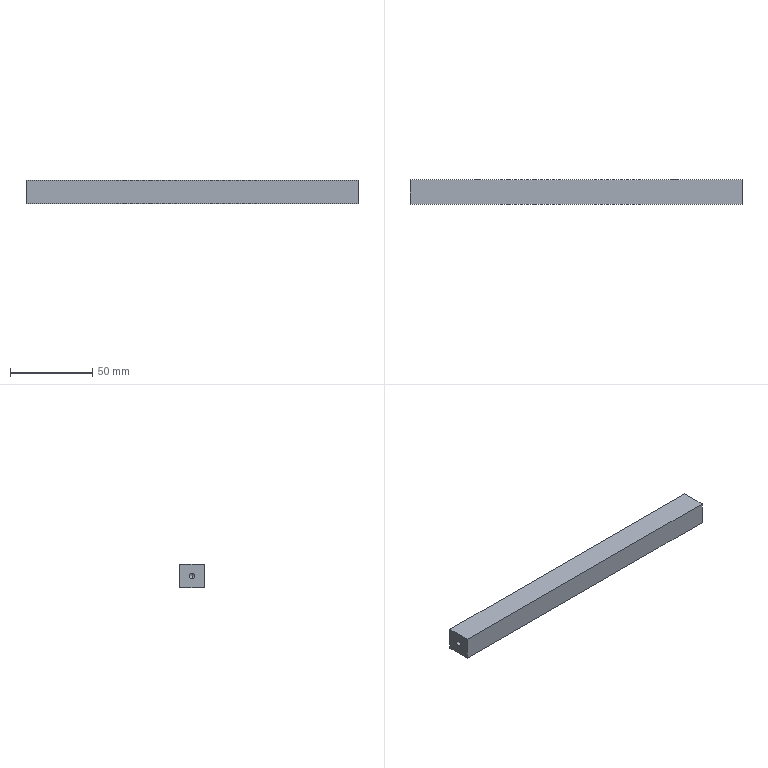CAM job | Mastercam | mm | 8 operations | part box 202 x 15 x 14
1. Facing | 12 - 12 平铣刀
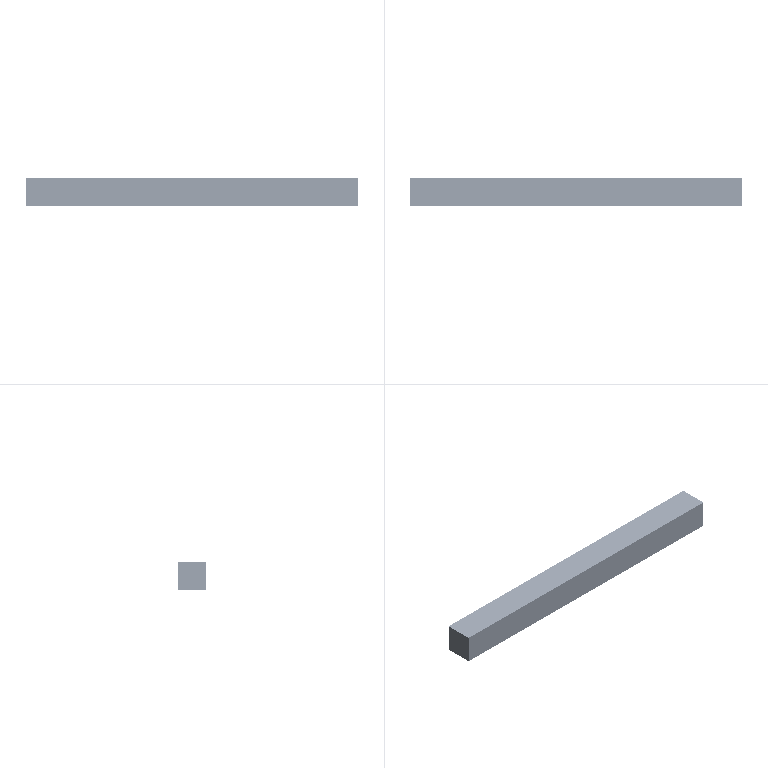2. 2D High Speed (2D Dynamic Mill) | 12 - 12 平铣刀
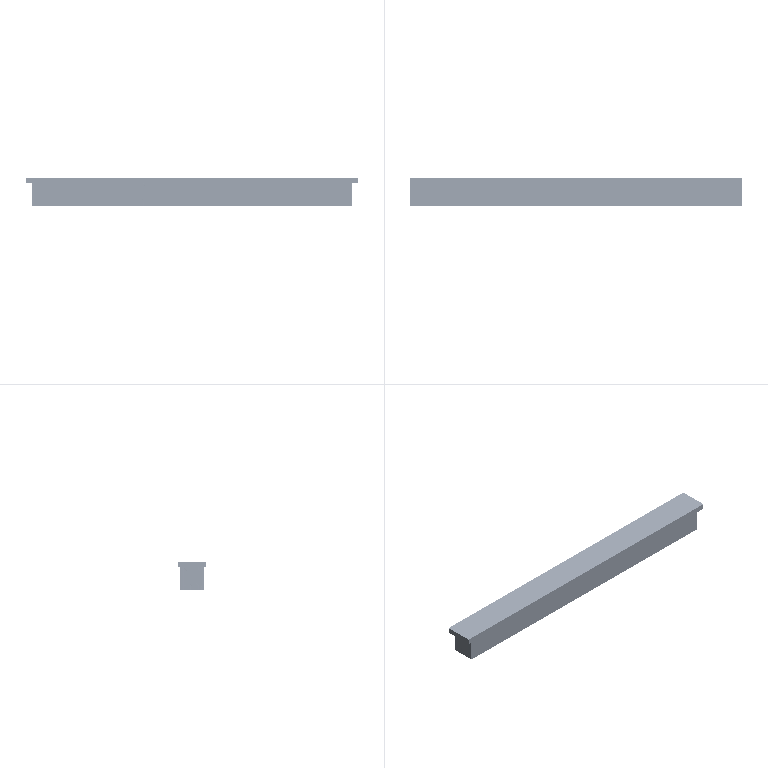3. Contour (2D) | 12 - 12 平铣刀
4. Model Chamfer | 7 - 4 倒角刀
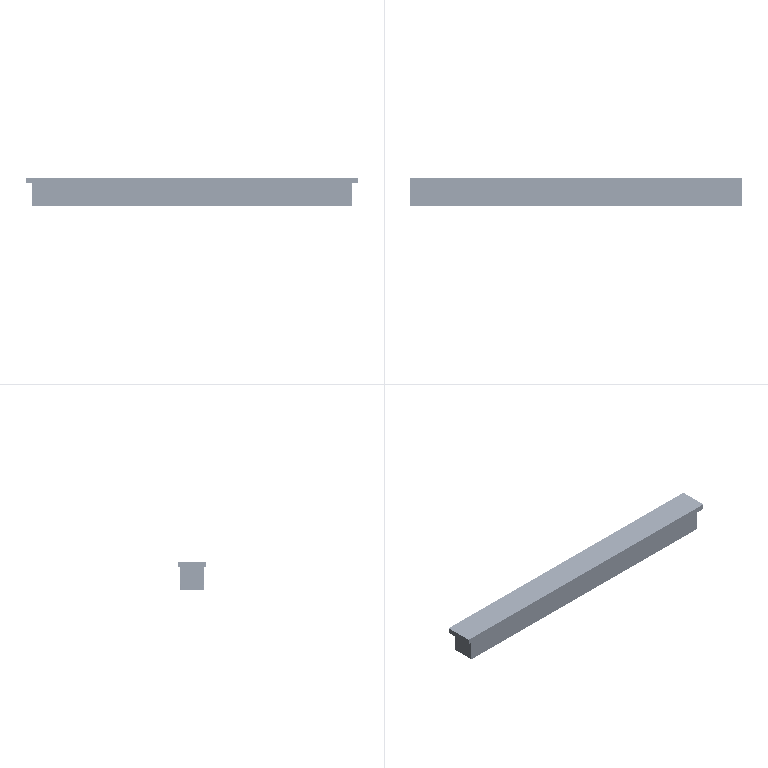5. Drill/Counterbore | 7 - 4 倒角刀
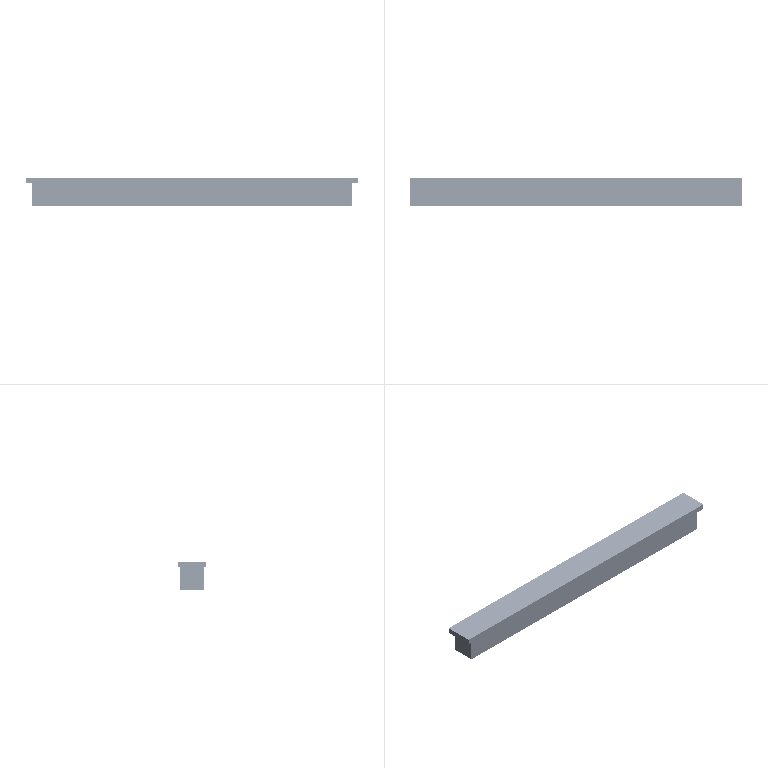6. Facing | 12 - 12 平铣刀
7. Contour (2D chamfer) | 7 - 4 倒角刀
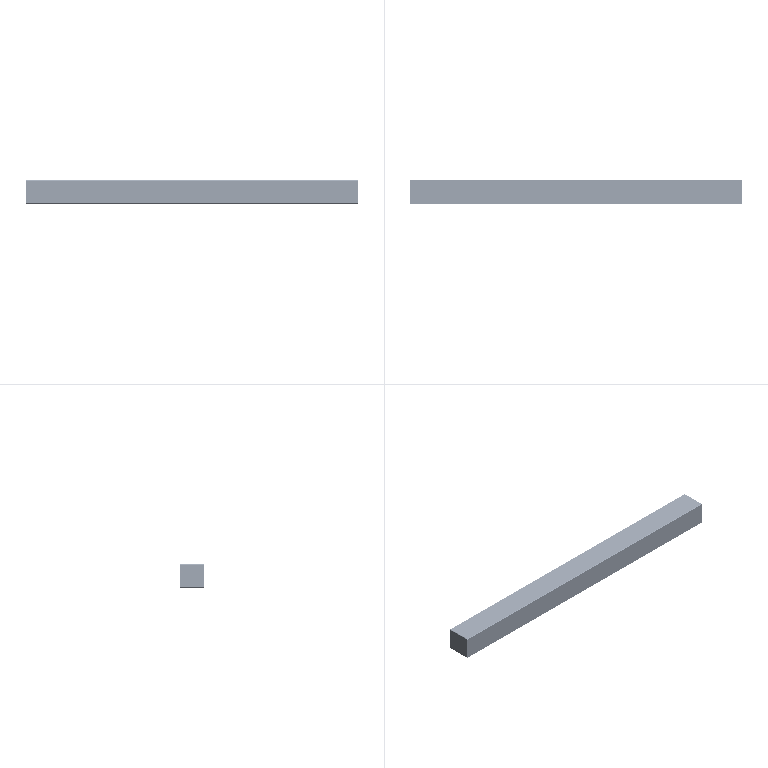8. Drill/Counterbore | 7 - 4 倒角刀